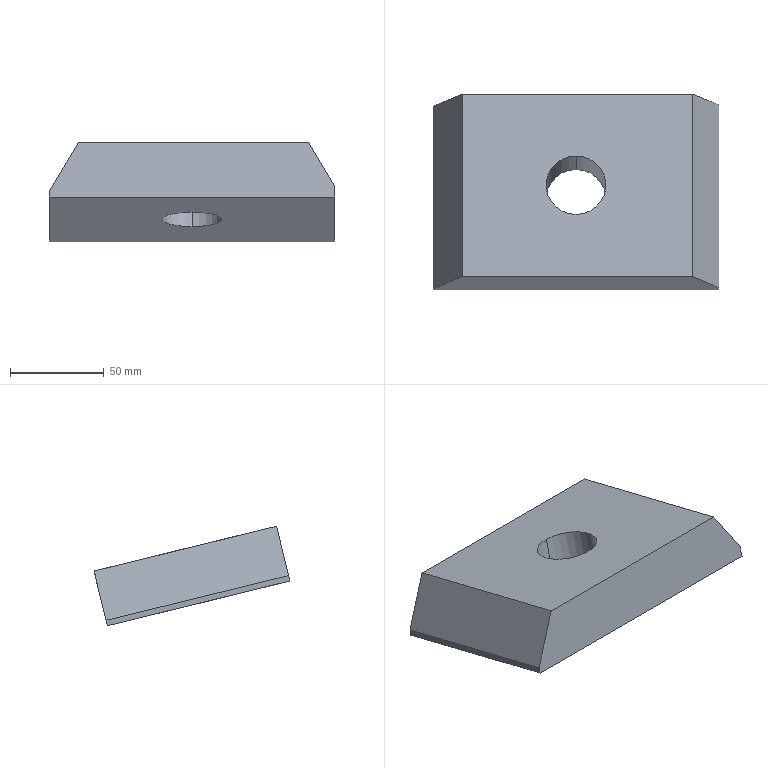Component | SolidWorks | Zatezna ploca-1 | 1 solid | 10 faces | box 152 x 104.27 x 52.92 mm | volume 393854 mm3 | plane 8 | cylinder 2 | commonest cylinder face diameters 32 x2
build123d program:
from build123d import *

# Parameters (mm, degrees)
BOSS_EXTRUDE1_DEPTH      = 1
BOSS_EXTRUDE1_DEPTH_BACK = 151
SKETCH1_W                = 30
SKETCH1_H                = 100
SKETCH2_R                = 16
CUT_EXTRUDE1_DEPTH       = 202.497
CHAMFER1_SIZE            = 27
CHAMFER1_SIZE2           = 15.588
CHAMFER2_SIZE            = 14
CHAMFER2_SIZE2           = 24.249


with BuildPart() as part:
    # Sketch1 → Boss-Extrude1 (new, two sides: drawn at the far end of the back side and taken through both)
    with BuildSketch(Plane.XY.offset(-BOSS_EXTRUDE1_DEPTH_BACK)):
        with Locations((-15, 80)):
            Rectangle(SKETCH1_W, SKETCH1_H)
    extrude(amount=BOSS_EXTRUDE1_DEPTH + BOSS_EXTRUDE1_DEPTH_BACK)

    # Sketch2 → Cut-Extrude1 (cut, through all)
    with BuildSketch(Plane(origin=(0, 0, 0), x_dir=(0, 0, -1), z_dir=(1, 0, 0))):
        with Locations(Location((75, 80, 0), (0, 0, 90))):
            Circle(SKETCH2_R)
    extrude(amount=-CUT_EXTRUDE1_DEPTH, mode=Mode.SUBTRACT)

    # Chamfer1
    chamfer1_edges = [part.edges().sort_by_distance(p)[0] for p in [
        (-30, 80, -151),
    ]]
    chamfer1_side = [part.faces().sort_by_distance(p)[0] for p in [
        (-15, 80, -151),
    ]]
    chamfer(chamfer1_edges, length=CHAMFER1_SIZE, length2=CHAMFER1_SIZE2, reference=chamfer1_side[0])

    # Chamfer2
    chamfer2_edges = [part.edges().sort_by_distance(p)[0] for p in [
        (-30, 80, 1),
    ]]
    chamfer2_side = [part.faces().sort_by_distance(p)[0] for p in [
        (-30, 128.309, -67.206),
    ]]
    chamfer(chamfer2_edges, length=CHAMFER2_SIZE, length2=CHAMFER2_SIZE2, reference=chamfer2_side[0])


solid = part.part

# Placed as in the assembly
solid = solid.moved(Location((0, 232.733, -101.11), (-13.755, 90, 0)))
STEP:
#1=COLOUR_RGB('',0.7922,0.8196,0.9333);
#2=FILL_AREA_STYLE_COLOUR('',#1);
#3=FILL_AREA_STYLE('',(#2));
#4=SURFACE_STYLE_FILL_AREA(#3);
#5=SURFACE_SIDE_STYLE('',(#4));
#6=SURFACE_STYLE_USAGE(.BOTH.,#5);
#7=PRESENTATION_STYLE_ASSIGNMENT((#6));
#8=CARTESIAN_POINT('',(-2.953,11.891,-3.433));
#9=VERTEX_POINT('',#8);
#10=CARTESIAN_POINT('',(-2.953,13.115,-3.732));
#11=VERTEX_POINT('',#10);
#12=CARTESIAN_POINT('',(-2.953,12.503,-3.582));
#13=DIRECTION('',(0.,-0.2378,-0.9713));
#14=DIRECTION('',(0.,0.9713,-0.2378));
#15=AXIS2_PLACEMENT_3D('',#12,#13,#14);
#16=CIRCLE('',#15,0.6299);
#17=EDGE_CURVE('',#9,#11,#16,.T.);
#18=ORIENTED_EDGE('',*,*,#17,.F.);
#19=CARTESIAN_POINT('',(-2.953,11.61,-4.58));
#20=VERTEX_POINT('',#19);
#21=CARTESIAN_POINT('',(-2.953,11.891,-3.433));
#22=DIRECTION('',(0.,-0.2378,-0.9713));
#23=VECTOR('',#22,39.37);
#24=LINE('',#21,#23);
#25=EDGE_CURVE('',#9,#20,#24,.T.);
#26=ORIENTED_EDGE('',*,*,#25,.T.);
#27=CARTESIAN_POINT('',(-2.953,12.834,-4.879));
#28=VERTEX_POINT('',#27);
#29=CARTESIAN_POINT('',(-2.953,12.222,-4.73));
#30=DIRECTION('',(0.,-0.2378,-0.9713));
#31=DIRECTION('',(0.,0.9713,-0.2378));
#32=AXIS2_PLACEMENT_3D('',#29,#30,#31);
#33=CIRCLE('',#32,0.6299);
#34=EDGE_CURVE('',#20,#28,#33,.T.);
#35=ORIENTED_EDGE('',*,*,#34,.T.);
#36=CARTESIAN_POINT('',(-2.953,13.115,-3.732));
#37=DIRECTION('',(0.,-0.2378,-0.9713));
#38=VECTOR('',#37,39.37);
#39=LINE('',#36,#38);
#40=EDGE_CURVE('',#11,#28,#39,.T.);
#41=ORIENTED_EDGE('',*,*,#40,.F.);
#42=EDGE_LOOP('',(#18,#26,#35,#41));
#43=FACE_OUTER_BOUND('',#42,.T.);
#44=CARTESIAN_POINT('',(-2.953,12.503,-3.582));
#45=DIRECTION('',(0.,-0.2378,-0.9713));
#46=DIRECTION('',(0.,0.9713,-0.2378));
#47=AXIS2_PLACEMENT_3D('',#44,#45,#46);
#48=CYLINDRICAL_SURFACE('',#47,0.6299);
#49=ADVANCED_FACE('',(#43),#48,.F.);
#50=CARTESIAN_POINT('',(-2.953,12.222,-4.73));
#51=DIRECTION('',(0.,-0.2378,-0.9713));
#52=DIRECTION('',(0.,0.9713,-0.2378));
#53=AXIS2_PLACEMENT_3D('',#50,#51,#52);
#54=CIRCLE('',#53,0.6299);
#55=EDGE_CURVE('',#28,#20,#54,.T.);
#56=ORIENTED_EDGE('',*,*,#55,.F.);
#57=ORIENTED_EDGE('',*,*,#34,.F.);
#58=EDGE_LOOP('',(#56,#57));
#59=FACE_BOUND('',#58,.T.);
#60=CARTESIAN_POINT('',(-5.945,14.134,-5.198));
#61=VERTEX_POINT('',#60);
#62=CARTESIAN_POINT('',(0.03937,14.134,-5.198));
#63=VERTEX_POINT('',#62);
#64=CARTESIAN_POINT('',(-5.945,14.134,-5.198));
#65=DIRECTION('',(1.,0.,0.));
#66=VECTOR('',#65,39.37);
#67=LINE('',#64,#66);
#68=EDGE_CURVE('',#61,#63,#67,.T.);
#69=ORIENTED_EDGE('',*,*,#68,.T.);
#70=CARTESIAN_POINT('',(0.03937,10.31,-4.262));
#71=VERTEX_POINT('',#70);
#72=CARTESIAN_POINT('',(0.03937,14.134,-5.198));
#73=DIRECTION('',(-0.,0.9713,-0.2378));
#74=VECTOR('',#73,39.37);
#75=LINE('',#72,#74);
#76=EDGE_CURVE('',#71,#63,#75,.T.);
#77=ORIENTED_EDGE('',*,*,#76,.F.);
#78=CARTESIAN_POINT('',(-5.945,10.31,-4.262));
#79=VERTEX_POINT('',#78);
#80=CARTESIAN_POINT('',(-5.945,10.31,-4.262));
#81=DIRECTION('',(1.,0.,0.));
#82=VECTOR('',#81,39.37);
#83=LINE('',#80,#82);
#84=EDGE_CURVE('',#79,#71,#83,.T.);
#85=ORIENTED_EDGE('',*,*,#84,.F.);
#86=CARTESIAN_POINT('',(-5.945,14.134,-5.198));
#87=DIRECTION('',(-0.,0.9713,-0.2378));
#88=VECTOR('',#87,39.37);
#89=LINE('',#86,#88);
#90=EDGE_CURVE('',#79,#61,#89,.T.);
#91=ORIENTED_EDGE('',*,*,#90,.T.);
#92=EDGE_LOOP('',(#69,#77,#85,#91));
#93=FACE_OUTER_BOUND('',#92,.T.);
#94=CARTESIAN_POINT('',(-5.945,14.134,-5.198));
#95=DIRECTION('',(0.,-0.2378,-0.9713));
#96=DIRECTION('',(-0.,0.9713,-0.2378));
#97=AXIS2_PLACEMENT_3D('',#94,#95,#96);
#98=PLANE('',#97);
#99=ADVANCED_FACE('',(#59,#93),#98,.T.);
#100=CARTESIAN_POINT('',(0.03937,10.364,-4.042));
#101=VERTEX_POINT('',#100);
#102=CARTESIAN_POINT('',(0.03937,10.31,-4.262));
#103=DIRECTION('',(0.,-0.2378,-0.9713));
#104=VECTOR('',#103,39.37);
#105=LINE('',#102,#104);
#106=EDGE_CURVE('',#101,#71,#105,.T.);
#107=ORIENTED_EDGE('',*,*,#106,.F.);
#108=CARTESIAN_POINT('',(-0.5118,10.591,-3.114));
#109=VERTEX_POINT('',#108);
#110=CARTESIAN_POINT('',(-1.359,10.94,-1.69));
#111=DIRECTION('',(-0.5,0.2059,0.8412));
#112=VECTOR('',#111,39.37);
#113=LINE('',#110,#112);
#114=EDGE_CURVE('',#101,#109,#113,.T.);
#115=ORIENTED_EDGE('',*,*,#114,.T.);
#116=CARTESIAN_POINT('',(-5.331,10.591,-3.114));
#117=VERTEX_POINT('',#116);
#118=CARTESIAN_POINT('',(-5.945,10.591,-3.114));
#119=DIRECTION('',(1.,0.,0.));
#120=VECTOR('',#119,39.37);
#121=LINE('',#118,#120);
#122=EDGE_CURVE('',#117,#109,#121,.T.);
#123=ORIENTED_EDGE('',*,*,#122,.F.);
#124=CARTESIAN_POINT('',(-5.945,10.338,-4.147));
#125=VERTEX_POINT('',#124);
#126=CARTESIAN_POINT('',(-5.996,10.317,-4.233));
#127=DIRECTION('',(-0.5,-0.2059,-0.8412));
#128=VECTOR('',#127,39.37);
#129=LINE('',#126,#128);
#130=EDGE_CURVE('',#117,#125,#129,.T.);
#131=ORIENTED_EDGE('',*,*,#130,.T.);
#132=CARTESIAN_POINT('',(-5.945,10.31,-4.262));
#133=DIRECTION('',(0.,-0.2378,-0.9713));
#134=VECTOR('',#133,39.37);
#135=LINE('',#132,#134);
#136=EDGE_CURVE('',#125,#79,#135,.T.);
#137=ORIENTED_EDGE('',*,*,#136,.T.);
#138=ORIENTED_EDGE('',*,*,#84,.T.);
#139=EDGE_LOOP('',(#107,#115,#123,#131,#137,#138));
#140=FACE_OUTER_BOUND('',#139,.T.);
#141=CARTESIAN_POINT('',(-5.945,10.31,-4.262));
#142=DIRECTION('',(0.,-0.9713,0.2378));
#143=DIRECTION('',(0.,-0.2378,-0.9713));
#144=AXIS2_PLACEMENT_3D('',#141,#142,#143);
#145=PLANE('',#144);
#146=ADVANCED_FACE('',(#140),#145,.T.);
#147=CARTESIAN_POINT('',(-2.953,12.503,-3.582));
#148=DIRECTION('',(0.,-0.2378,-0.9713));
#149=DIRECTION('',(0.,0.9713,-0.2378));
#150=AXIS2_PLACEMENT_3D('',#147,#148,#149);
#151=CIRCLE('',#150,0.6299);
#152=EDGE_CURVE('',#11,#9,#151,.T.);
#153=ORIENTED_EDGE('',*,*,#152,.T.);
#154=ORIENTED_EDGE('',*,*,#17,.T.);
#155=EDGE_LOOP('',(#153,#154));
#156=FACE_BOUND('',#155,.T.);
#157=ORIENTED_EDGE('',*,*,#122,.T.);
#158=CARTESIAN_POINT('',(-0.5118,14.415,-4.05));
#159=VERTEX_POINT('',#158);
#160=CARTESIAN_POINT('',(-0.5118,14.415,-4.05));
#161=DIRECTION('',(-0.,0.9713,-0.2378));
#162=VECTOR('',#161,39.37);
#163=LINE('',#160,#162);
#164=EDGE_CURVE('',#109,#159,#163,.T.);
#165=ORIENTED_EDGE('',*,*,#164,.T.);
#166=CARTESIAN_POINT('',(-5.331,14.415,-4.05));
#167=VERTEX_POINT('',#166);
#168=CARTESIAN_POINT('',(-5.945,14.415,-4.05));
#169=DIRECTION('',(1.,0.,0.));
#170=VECTOR('',#169,39.37);
#171=LINE('',#168,#170);
#172=EDGE_CURVE('',#167,#159,#171,.T.);
#173=ORIENTED_EDGE('',*,*,#172,.F.);
#174=CARTESIAN_POINT('',(-5.331,14.415,-4.05));
#175=DIRECTION('',(0.,-0.9713,0.2378));
#176=VECTOR('',#175,39.37);
#177=LINE('',#174,#176);
#178=EDGE_CURVE('',#167,#117,#177,.T.);
#179=ORIENTED_EDGE('',*,*,#178,.T.);
#180=EDGE_LOOP('',(#157,#165,#173,#179));
#181=FACE_OUTER_BOUND('',#180,.T.);
#182=CARTESIAN_POINT('',(-5.945,14.415,-4.05));
#183=DIRECTION('',(-0.,0.2378,0.9713));
#184=DIRECTION('',(0.,-0.9713,0.2378));
#185=AXIS2_PLACEMENT_3D('',#182,#183,#184);
#186=PLANE('',#185);
#187=ADVANCED_FACE('',(#156,#181),#186,.T.);
#188=ORIENTED_EDGE('',*,*,#172,.T.);
#189=CARTESIAN_POINT('',(0.03937,14.188,-4.978));
#190=VERTEX_POINT('',#189);
#191=CARTESIAN_POINT('',(-1.359,14.764,-2.626));
#192=DIRECTION('',(0.5,-0.2059,-0.8412));
#193=VECTOR('',#192,39.37);
#194=LINE('',#191,#193);
#195=EDGE_CURVE('',#159,#190,#194,.T.);
#196=ORIENTED_EDGE('',*,*,#195,.T.);
#197=CARTESIAN_POINT('',(0.03937,14.134,-5.198));
#198=DIRECTION('',(-0.,0.2378,0.9713));
#199=VECTOR('',#198,39.37);
#200=LINE('',#197,#199);
#201=EDGE_CURVE('',#63,#190,#200,.T.);
#202=ORIENTED_EDGE('',*,*,#201,.F.);
#203=ORIENTED_EDGE('',*,*,#68,.F.);
#204=CARTESIAN_POINT('',(-5.945,14.162,-5.083));
#205=VERTEX_POINT('',#204);
#206=CARTESIAN_POINT('',(-5.945,14.134,-5.198));
#207=DIRECTION('',(-0.,0.2378,0.9713));
#208=VECTOR('',#207,39.37);
#209=LINE('',#206,#208);
#210=EDGE_CURVE('',#61,#205,#209,.T.);
#211=ORIENTED_EDGE('',*,*,#210,.T.);
#212=CARTESIAN_POINT('',(-5.996,14.141,-5.169));
#213=DIRECTION('',(0.5,0.2059,0.8412));
#214=VECTOR('',#213,39.37);
#215=LINE('',#212,#214);
#216=EDGE_CURVE('',#205,#167,#215,.T.);
#217=ORIENTED_EDGE('',*,*,#216,.T.);
#218=EDGE_LOOP('',(#188,#196,#202,#203,#211,#217));
#219=FACE_OUTER_BOUND('',#218,.T.);
#220=CARTESIAN_POINT('',(-5.945,14.134,-5.198));
#221=DIRECTION('',(-0.,0.9713,-0.2378));
#222=DIRECTION('',(1.,0.,0.));
#223=AXIS2_PLACEMENT_3D('',#220,#221,#222);
#224=PLANE('',#223);
#225=ADVANCED_FACE('',(#219),#224,.T.);
#226=ORIENTED_EDGE('',*,*,#136,.F.);
#227=CARTESIAN_POINT('',(-5.945,9.191,-3.866));
#228=DIRECTION('',(-0.,0.9713,-0.2378));
#229=VECTOR('',#228,39.37);
#230=LINE('',#227,#229);
#231=EDGE_CURVE('',#125,#205,#230,.T.);
#232=ORIENTED_EDGE('',*,*,#231,.T.);
#233=ORIENTED_EDGE('',*,*,#210,.F.);
#234=ORIENTED_EDGE('',*,*,#90,.F.);
#235=EDGE_LOOP('',(#226,#232,#233,#234));
#236=FACE_OUTER_BOUND('',#235,.T.);
#237=CARTESIAN_POINT('',(-5.945,9.163,-3.981));
#238=DIRECTION('',(-1.,-0.,0.));
#239=DIRECTION('',(-0.,0.2378,0.9713));
#240=AXIS2_PLACEMENT_3D('',#237,#238,#239);
#241=PLANE('',#240);
#242=ADVANCED_FACE('',(#236),#241,.T.);
#243=ORIENTED_EDGE('',*,*,#201,.T.);
#244=CARTESIAN_POINT('',(0.03937,10.364,-4.042));
#245=DIRECTION('',(0.,-0.9713,0.2378));
#246=VECTOR('',#245,39.37);
#247=LINE('',#244,#246);
#248=EDGE_CURVE('',#190,#101,#247,.T.);
#249=ORIENTED_EDGE('',*,*,#248,.T.);
#250=ORIENTED_EDGE('',*,*,#106,.T.);
#251=ORIENTED_EDGE('',*,*,#76,.T.);
#252=EDGE_LOOP('',(#243,#249,#250,#251));
#253=FACE_OUTER_BOUND('',#252,.T.);
#254=CARTESIAN_POINT('',(0.03937,9.163,-3.981));
#255=DIRECTION('',(-1.,-0.,0.));
#256=DIRECTION('',(-0.,0.2378,0.9713));
#257=AXIS2_PLACEMENT_3D('',#254,#255,#256);
#258=PLANE('',#257);
#259=ADVANCED_FACE('',(#253),#258,.F.);
#260=ORIENTED_EDGE('',*,*,#25,.F.);
#261=ORIENTED_EDGE('',*,*,#152,.F.);
#262=ORIENTED_EDGE('',*,*,#40,.T.);
#263=ORIENTED_EDGE('',*,*,#55,.T.);
#264=EDGE_LOOP('',(#260,#261,#262,#263));
#265=FACE_OUTER_BOUND('',#264,.T.);
#266=CARTESIAN_POINT('',(-2.953,12.503,-3.582));
#267=DIRECTION('',(0.,-0.2378,-0.9713));
#268=DIRECTION('',(0.,0.9713,-0.2378));
#269=AXIS2_PLACEMENT_3D('',#266,#267,#268);
#270=CYLINDRICAL_SURFACE('',#269,0.6299);
#271=ADVANCED_FACE('',(#265),#270,.F.);
#272=ORIENTED_EDGE('',*,*,#216,.F.);
#273=ORIENTED_EDGE('',*,*,#231,.F.);
#274=ORIENTED_EDGE('',*,*,#130,.F.);
#275=ORIENTED_EDGE('',*,*,#178,.F.);
#276=EDGE_LOOP('',(#272,#273,#274,#275));
#277=FACE_OUTER_BOUND('',#276,.T.);
#278=CARTESIAN_POINT('',(-5.331,14.415,-4.05));
#279=DIRECTION('',(0.866,-0.1189,-0.4857));
#280=DIRECTION('',(0.,-0.9713,0.2378));
#281=AXIS2_PLACEMENT_3D('',#278,#279,#280);
#282=PLANE('',#281);
#283=ADVANCED_FACE('',(#277),#282,.F.);
#284=ORIENTED_EDGE('',*,*,#195,.F.);
#285=ORIENTED_EDGE('',*,*,#164,.F.);
#286=ORIENTED_EDGE('',*,*,#114,.F.);
#287=ORIENTED_EDGE('',*,*,#248,.F.);
#288=EDGE_LOOP('',(#284,#285,#286,#287));
#289=FACE_OUTER_BOUND('',#288,.T.);
#290=CARTESIAN_POINT('',(0.03937,9.217,-3.761));
#291=DIRECTION('',(0.866,0.1189,0.4857));
#292=DIRECTION('',(-0.,0.9713,-0.2378));
#293=AXIS2_PLACEMENT_3D('',#290,#291,#292);
#294=PLANE('',#293);
#295=ADVANCED_FACE('',(#289),#294,.T.);
#296=CLOSED_SHELL('',(#49,#99,#146,#187,#225,#242,#259,#271,#283,#295));
#297=MANIFOLD_SOLID_BREP('',#296);
#298=STYLED_ITEM('',(#7),#297);
#299=PRESENTATION_LAYER_ASSIGNMENT('','',(#298));
#300=(LENGTH_UNIT()NAMED_UNIT(*)SI_UNIT($,.METRE.));
#301=LENGTH_MEASURE_WITH_UNIT(LENGTH_MEASURE(0.0254),#300);
#302=DIMENSIONAL_EXPONENTS(1.,0.,0.,0.,0.,0.,0.);
#303=(CONVERSION_BASED_UNIT('',#301)LENGTH_UNIT()NAMED_UNIT(#302));
#304=UNCERTAINTY_MEASURE_WITH_UNIT(LENGTH_MEASURE(0.00001),#303,'','');
#305=(NAMED_UNIT(*)PLANE_ANGLE_UNIT()SI_UNIT($,.RADIAN.));
#306=(NAMED_UNIT(*)SI_UNIT($,.STERADIAN.)SOLID_ANGLE_UNIT());
#307=(GEOMETRIC_REPRESENTATION_CONTEXT(3)GLOBAL_UNCERTAINTY_ASSIGNED_CONTEXT((#304))GLOBAL_UNIT_ASSIGNED_CONTEXT((#303,#305,#306))REPRESENTATION_CONTEXT('',''));
#308=MECHANICAL_DESIGN_GEOMETRIC_PRESENTATION_REPRESENTATION('',(#298),#307);
#309=CARTESIAN_POINT('',(0.,0.,0.));
#310=DIRECTION('',(0.,0.,1.));
#311=DIRECTION('',(1.,0.,0.));
#312=AXIS2_PLACEMENT_3D('',#309,#310,#311);
#313=(LENGTH_UNIT()NAMED_UNIT(*)SI_UNIT($,.METRE.));
#314=LENGTH_MEASURE_WITH_UNIT(LENGTH_MEASURE(0.0254),#313);
#315=DIMENSIONAL_EXPONENTS(1.,0.,0.,0.,0.,0.,0.);
#316=(CONVERSION_BASED_UNIT('',#314)LENGTH_UNIT()NAMED_UNIT(#315));
#317=UNCERTAINTY_MEASURE_WITH_UNIT(LENGTH_MEASURE(0.00001),#316,'','');
#318=(NAMED_UNIT(*)PLANE_ANGLE_UNIT()SI_UNIT($,.RADIAN.));
#319=(NAMED_UNIT(*)SI_UNIT($,.STERADIAN.)SOLID_ANGLE_UNIT());
#320=(GEOMETRIC_REPRESENTATION_CONTEXT(3)GLOBAL_UNCERTAINTY_ASSIGNED_CONTEXT((#317))GLOBAL_UNIT_ASSIGNED_CONTEXT((#316,#318,#319))REPRESENTATION_CONTEXT('',''));
#321=ADVANCED_BREP_SHAPE_REPRESENTATION('',(#297,#312),#320);